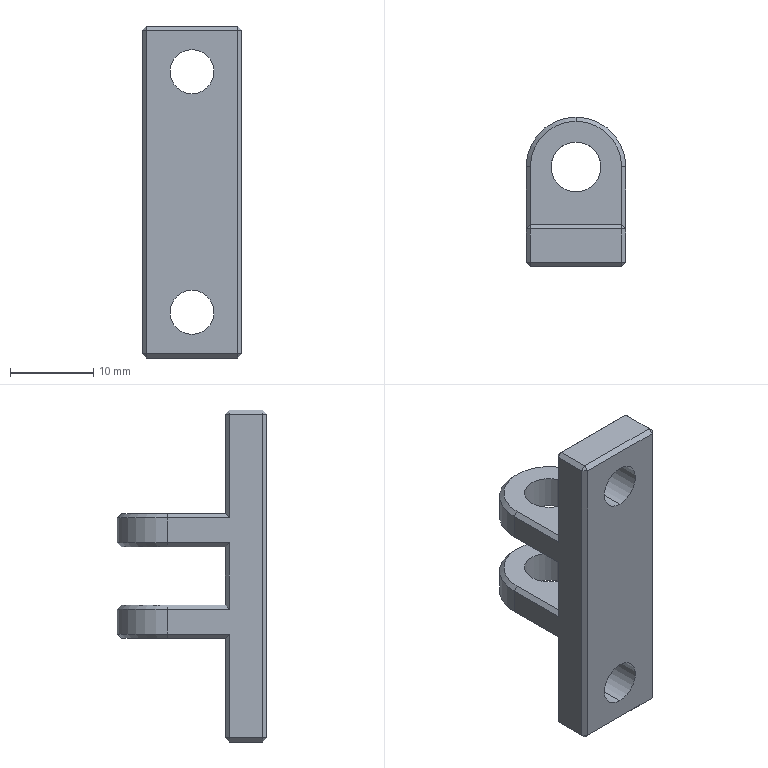Part | SolidWorks | mm | 1 solid | 64 faces | box 12 x 18 x 40 mm | volume 3035 mm3 | plane 44 | cylinder 12 | cone 8 | commonest cylinder face diameters 6 x4 5.3 x4 12 x4